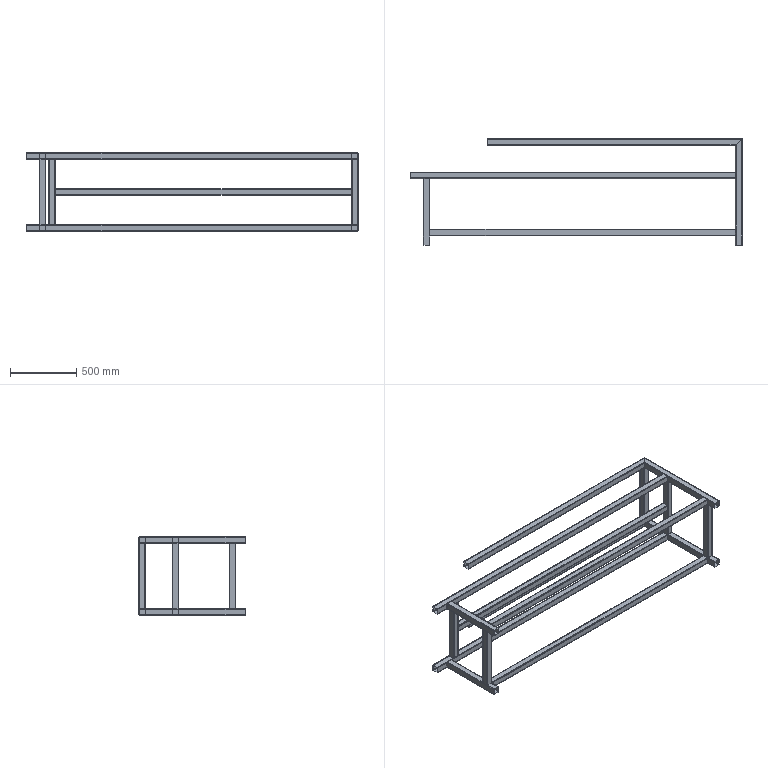Component | SolidWorks | Frame-1 | 16 solids | 288 faces | box 2500 x 800 x 590 mm | volume 9415617 mm3 | plane 160 | cylinder 128 | commonest cylinder face diameters 5 x64 10 x64
build123d program:
from build123d import *

# Parameters (mm, degrees)
SQUARE_TUBE_50_X_50_X_2_5_1_DEPTH     = 526
SQUARE_TUBE_50_X_50_X_2_5_1_2_DEPTH   = 775
SQUARE_TUBE_50_X_50_X_2_5_1_3_DEPTH   = 2352
SQUARE_TUBE_50_X_50_X_2_5_1_4_DEPTH   = 2476
SQUARE_TUBE_50_X_50_X_2_5_2_DEPTH     = 1895
BODY_START                            = 141.421
BODY_5_RUN_ON_DEPTH                   = 166.421
BODY_START_2                          = 633.579
BODY_2_RUN_ON_DEPTH                   = 166.421
SQUARE_TUBE_50_X_50_X_2_5_5_DEPTH     = 526
SQUARE_TUBE_50_X_50_X_2_5_5_2_DEPTH   = 800
SQUARE_TUBE_50_X_50_X_2_5_5_3_DEPTH   = 2352
SQUARE_TUBE_50_X_50_X_2_5_5_4_DEPTH   = 2476
SQUARE_TUBE_50_X_50_X_2_5_5_5_DEPTH   = 1896
BODY_START_3                          = 167.421
BODY_10_RUN_ON_DEPTH                  = 191.421
SQUARE_TUBE_50_X_50_X_2_5_6_DEPTH     = 540
SQUARE_TUBE_50_X_50_X_2_5_6_2_DEPTH   = 540
SQUARE_TUBE_50_X_50_X_2_5_6_3_DEPTH   = 540
SQUARE_TUBE_50_X_50_X_2_5_6_4_DEPTH   = 540
SQUARE_TUBE_50_X_50_X_2_5_6_5_DEPTH   = 540
SQUARE_TUBE_50_X_50_X_2_5_1_2_2_DEPTH = 2277.579


with BuildPart() as part:
    # Sketch1 → Square Tube 50 X 50 X 2.5_1 (new body)
    with BuildSketch(Plane(origin=(0, 0, 0), x_dir=(1, 0, 0), z_dir=(0, 1, 0))):
        with BuildLine():
            Line((-20, -25), (20, -25))
            ThreePointArc((20, -25), (23.536, -23.536), (25, -20))
            Line((25, -20), (25, 20))
            ThreePointArc((25, 20), (23.536, 23.536), (20, 25))
            Line((20, 25), (-20, 25))
            ThreePointArc((-20, 25), (-23.536, 23.536), (-25, 20))
            Line((-25, 20), (-25, -20))
            ThreePointArc((-25, -20), (-23.536, -23.536), (-20, -25))
        make_face()
        with BuildLine():
            Line((-20, -22.5), (20, -22.5))
            ThreePointArc((20, -22.5), (21.768, -21.768), (22.5, -20))
            Line((22.5, -20), (22.5, 20))
            ThreePointArc((22.5, 20), (21.768, 21.768), (20, 22.5))
            Line((20, 22.5), (-20, 22.5))
            ThreePointArc((-20, 22.5), (-21.768, 21.768), (-22.5, 20))
            Line((-22.5, 20), (-22.5, -20))
            ThreePointArc((-22.5, -20), (-21.768, -21.768), (-20, -22.5))
        make_face(mode=Mode.SUBTRACT)
    extrude(amount=SQUARE_TUBE_50_X_50_X_2_5_1_DEPTH)

    # Square Tube 50 X 50 X 2.5_1 end butt 1
    split(bisect_by=Plane.XZ.offset(-500), keep=Keep.TOP)


with BuildPart() as body_2:
    # Sketch1 on segment 2 (on carried to segment 2) → Square Tube 50 X 50 X 2.5_1 2 (new body)
    with BuildSketch(Plane(origin=(2350, 0, 0), x_dir=(1, 0, 0), z_dir=(0, 1, 0))):
        with BuildLine():
            Line((-20, -25), (20, -25))
            ThreePointArc((20, -25), (23.536, -23.536), (25, -20))
            Line((25, -20), (25, 20))
            ThreePointArc((25, 20), (23.536, 23.536), (20, 25))
            Line((20, 25), (-20, 25))
            ThreePointArc((-20, 25), (-23.536, 23.536), (-25, 20))
            Line((-25, 20), (-25, -20))
            ThreePointArc((-25, -20), (-23.536, -23.536), (-20, -25))
        make_face()
        with BuildLine():
            Line((-20, -22.5), (20, -22.5))
            ThreePointArc((20, -22.5), (21.768, -21.768), (22.5, -20))
            Line((22.5, -20), (22.5, 20))
            ThreePointArc((22.5, 20), (21.768, 21.768), (20, 22.5))
            Line((20, 22.5), (-20, 22.5))
            ThreePointArc((-20, 22.5), (-21.768, 21.768), (-22.5, 20))
            Line((-22.5, 20), (-22.5, -20))
            ThreePointArc((-22.5, -20), (-21.768, -21.768), (-20, -22.5))
        make_face(mode=Mode.SUBTRACT)
    extrude(amount=SQUARE_TUBE_50_X_50_X_2_5_1_2_DEPTH)

    # body 2 cut square before the run-on
    split(bisect_by=Plane(origin=(2350, 633.579, 0), x_dir=(1, 0, 0), z_dir=(0, -1, 0)), keep=Keep.TOP)

    # Sketch1 on segment 2 (on carried to segment 2) → body 2 run on (add)
    with BuildSketch(Plane(origin=(2350, 0, 0), x_dir=(1, 0, 0), z_dir=(0, 1, 0)).offset(BODY_START_2)):
        with BuildLine():
            Line((-20, -25), (20, -25))
            ThreePointArc((20, -25), (23.536, -23.536), (25, -20))
            Line((25, -20), (25, 20))
            ThreePointArc((25, 20), (23.536, 23.536), (20, 25))
            Line((20, 25), (-20, 25))
            ThreePointArc((-20, 25), (-23.536, 23.536), (-25, 20))
            Line((-25, 20), (-25, -20))
            ThreePointArc((-25, -20), (-23.536, -23.536), (-20, -25))
        make_face()
        with BuildLine():
            Line((-20, -22.5), (20, -22.5))
            ThreePointArc((20, -22.5), (21.768, -21.768), (22.5, -20))
            Line((22.5, -20), (22.5, 20))
            ThreePointArc((22.5, 20), (21.768, 21.768), (20, 22.5))
            Line((20, 22.5), (-20, 22.5))
            ThreePointArc((-20, 22.5), (-21.768, 21.768), (-22.5, 20))
            Line((-22.5, 20), (-22.5, -20))
            ThreePointArc((-22.5, -20), (-21.768, -21.768), (-20, -22.5))
        make_face(mode=Mode.SUBTRACT)
    extrude(amount=BODY_2_RUN_ON_DEPTH)

    # Trim_Extend1
    split(bisect_by=Plane(origin=(2350, 775, 0), x_dir=(0.7071, 0.7071, 0), z_dir=(0.7071, -0.7071, 0)), keep=Keep.TOP)


with BuildPart() as body_3:
    # Sketch1 on segment 3 (on carried to segment 3) → Square Tube 50 X 50 X 2.5_1 3 (new body)
    with BuildSketch(Plane(origin=(-1, 95, 0), x_dir=(0, -1, 0), z_dir=(1, 0, 0))):
        with BuildLine():
            Line((-20, -25), (20, -25))
            ThreePointArc((20, -25), (23.536, -23.536), (25, -20))
            Line((25, -20), (25, 20))
            ThreePointArc((25, 20), (23.536, 23.536), (20, 25))
            Line((20, 25), (-20, 25))
            ThreePointArc((-20, 25), (-23.536, 23.536), (-25, 20))
            Line((-25, 20), (-25, -20))
            ThreePointArc((-25, -20), (-23.536, -23.536), (-20, -25))
        make_face()
        with BuildLine():
            Line((-20, -22.5), (20, -22.5))
            ThreePointArc((20, -22.5), (21.768, -21.768), (22.5, -20))
            Line((22.5, -20), (22.5, 20))
            ThreePointArc((22.5, 20), (21.768, 21.768), (20, 22.5))
            Line((20, 22.5), (-20, 22.5))
            ThreePointArc((-20, 22.5), (-21.768, 21.768), (-22.5, 20))
            Line((-22.5, 20), (-22.5, -20))
            ThreePointArc((-22.5, -20), (-21.768, -21.768), (-20, -22.5))
        make_face(mode=Mode.SUBTRACT)
    extrude(amount=SQUARE_TUBE_50_X_50_X_2_5_1_3_DEPTH)

    # Square Tube 50 X 50 X 2.5_1 3 end butt 1
    split(bisect_by=Plane(origin=(25, 95, 0), x_dir=(0, 1, 0), z_dir=(1, 0, 0)), keep=Keep.TOP)

    # Square Tube 50 X 50 X 2.5_1 3 end butt 2
    split(bisect_by=Plane(origin=(2325, 95, 0), x_dir=(0, -1, 0), z_dir=(-1, 0, 0)), keep=Keep.TOP)


with BuildPart() as body_4:
    # Sketch1 on segment 4 (on carried to segment 4) → Square Tube 50 X 50 X 2.5_1 4 (new body)
    with BuildSketch(Plane(origin=(-125, 525, 0), x_dir=(0, -1, 0), z_dir=(1, 0, 0))):
        with BuildLine():
            Line((-20, -25), (20, -25))
            ThreePointArc((20, -25), (23.536, -23.536), (25, -20))
            Line((25, -20), (25, 20))
            ThreePointArc((25, 20), (23.536, 23.536), (20, 25))
            Line((20, 25), (-20, 25))
            ThreePointArc((-20, 25), (-23.536, 23.536), (-25, 20))
            Line((-25, 20), (-25, -20))
            ThreePointArc((-25, -20), (-23.536, -23.536), (-20, -25))
        make_face()
        with BuildLine():
            Line((-20, -22.5), (20, -22.5))
            ThreePointArc((20, -22.5), (21.768, -21.768), (22.5, -20))
            Line((22.5, -20), (22.5, 20))
            ThreePointArc((22.5, 20), (21.768, 21.768), (20, 22.5))
            Line((20, 22.5), (-20, 22.5))
            ThreePointArc((-20, 22.5), (-21.768, 21.768), (-22.5, 20))
            Line((-22.5, 20), (-22.5, -20))
            ThreePointArc((-22.5, -20), (-21.768, -21.768), (-20, -22.5))
        make_face(mode=Mode.SUBTRACT)
    extrude(amount=SQUARE_TUBE_50_X_50_X_2_5_1_4_DEPTH)

    # Square Tube 50 X 50 X 2.5_1 4 end butt 1
    split(bisect_by=Plane(origin=(2325, 525, 0), x_dir=(0, -1, 0), z_dir=(-1, 0, 0)), keep=Keep.TOP)


with BuildPart() as body_5:
    # Sketch11 → Square Tube 50 X 50 X 2.5_2 (new body)
    with BuildSketch(Plane(origin=(2350, 775, 0), x_dir=(0, 0, 1), z_dir=(-1, 0, 0))):
        with BuildLine():
            Line((-20, -25), (20, -25))
            ThreePointArc((20, -25), (23.536, -23.536), (25, -20))
            Line((25, -20), (25, 20))
            ThreePointArc((25, 20), (23.536, 23.536), (20, 25))
            Line((20, 25), (-20, 25))
            ThreePointArc((-20, 25), (-23.536, 23.536), (-25, 20))
            Line((-25, 20), (-25, -20))
            ThreePointArc((-25, -20), (-23.536, -23.536), (-20, -25))
        make_face()
        with BuildLine():
            Line((-20, -22.5), (20, -22.5))
            ThreePointArc((20, -22.5), (21.768, -21.768), (22.5, -20))
            Line((22.5, -20), (22.5, 20))
            ThreePointArc((22.5, 20), (21.768, 21.768), (20, 22.5))
            Line((20, 22.5), (-20, 22.5))
            ThreePointArc((-20, 22.5), (-21.768, 21.768), (-22.5, 20))
            Line((-22.5, 20), (-22.5, -20))
            ThreePointArc((-22.5, -20), (-21.768, -21.768), (-20, -22.5))
        make_face(mode=Mode.SUBTRACT)
    extrude(amount=SQUARE_TUBE_50_X_50_X_2_5_2_DEPTH)

    # body 5 cut square before the run-on
    split(bisect_by=Plane(origin=(2208.579, 775, 0), x_dir=(0, -1, 0), z_dir=(-1, 0, 0)), keep=Keep.TOP)

    # Sketch11 → body 5 run on (add)
    with BuildSketch(Plane(origin=(2350, 775, 0), x_dir=(0, 0, 1), z_dir=(-1, 0, 0)).offset(BODY_START)):
        with BuildLine():
            Line((-20, -25), (20, -25))
            ThreePointArc((20, -25), (23.536, -23.536), (25, -20))
            Line((25, -20), (25, 20))
            ThreePointArc((25, 20), (23.536, 23.536), (20, 25))
            Line((20, 25), (-20, 25))
            ThreePointArc((-20, 25), (-23.536, 23.536), (-25, 20))
            Line((-25, 20), (-25, -20))
            ThreePointArc((-25, -20), (-23.536, -23.536), (-20, -25))
        make_face()
        with BuildLine():
            Line((-20, -22.5), (20, -22.5))
            ThreePointArc((20, -22.5), (21.768, -21.768), (22.5, -20))
            Line((22.5, -20), (22.5, 20))
            ThreePointArc((22.5, 20), (21.768, 21.768), (20, 22.5))
            Line((20, 22.5), (-20, 22.5))
            ThreePointArc((-20, 22.5), (-21.768, 21.768), (-22.5, 20))
            Line((-22.5, 20), (-22.5, -20))
            ThreePointArc((-22.5, -20), (-21.768, -21.768), (-20, -22.5))
        make_face(mode=Mode.SUBTRACT)
    extrude(amount=-BODY_5_RUN_ON_DEPTH)

    # Trim_Extend1
    split(bisect_by=Plane(origin=(2350, 775, 0), x_dir=(-0.7071, -0.7071, 0), z_dir=(-0.7071, 0.7071, 0)), keep=Keep.TOP)


with BuildPart() as body_6:
    # Sketch12 → Square Tube 50 X 50 X 2.5_5 (new body)
    with BuildSketch(Plane(origin=(0, 0, 540), x_dir=(-1, 0, 0), z_dir=(0, 1, 0))):
        with BuildLine():
            Line((-20, -25), (20, -25))
            ThreePointArc((20, -25), (23.536, -23.536), (25, -20))
            Line((25, -20), (25, 20))
            ThreePointArc((25, 20), (23.536, 23.536), (20, 25))
            Line((20, 25), (-20, 25))
            ThreePointArc((-20, 25), (-23.536, 23.536), (-25, 20))
            Line((-25, 20), (-25, -20))
            ThreePointArc((-25, -20), (-23.536, -23.536), (-20, -25))
        make_face()
        with BuildLine():
            Line((-20, -22.5), (20, -22.5))
            ThreePointArc((20, -22.5), (21.768, -21.768), (22.5, -20))
            Line((22.5, -20), (22.5, 20))
            ThreePointArc((22.5, 20), (21.768, 21.768), (20, 22.5))
            Line((20, 22.5), (-20, 22.5))
            ThreePointArc((-20, 22.5), (-21.768, 21.768), (-22.5, 20))
            Line((-22.5, 20), (-22.5, -20))
            ThreePointArc((-22.5, -20), (-21.768, -21.768), (-20, -22.5))
        make_face(mode=Mode.SUBTRACT)
    extrude(amount=SQUARE_TUBE_50_X_50_X_2_5_5_DEPTH)

    # Square Tube 50 X 50 X 2.5_5 end butt 1
    split(bisect_by=Plane(origin=(0, 500, 540), x_dir=(1, 0, 0), z_dir=(0, -1, 0)), keep=Keep.TOP)


with BuildPart() as body_7:
    # Sketch12 on segment 2 (on carried to segment 2) → Square Tube 50 X 50 X 2.5_5 2 (new body)
    with BuildSketch(Plane(origin=(2350, 0, 540), x_dir=(-1, 0, 0), z_dir=(0, 1, 0))):
        with BuildLine():
            Line((-20, -25), (20, -25))
            ThreePointArc((20, -25), (23.536, -23.536), (25, -20))
            Line((25, -20), (25, 20))
            ThreePointArc((25, 20), (23.536, 23.536), (20, 25))
            Line((20, 25), (-20, 25))
            ThreePointArc((-20, 25), (-23.536, 23.536), (-25, 20))
            Line((-25, 20), (-25, -20))
            ThreePointArc((-25, -20), (-23.536, -23.536), (-20, -25))
        make_face()
        with BuildLine():
            Line((-20, -22.5), (20, -22.5))
            ThreePointArc((20, -22.5), (21.768, -21.768), (22.5, -20))
            Line((22.5, -20), (22.5, 20))
            ThreePointArc((22.5, 20), (21.768, 21.768), (20, 22.5))
            Line((20, 22.5), (-20, 22.5))
            ThreePointArc((-20, 22.5), (-21.768, 21.768), (-22.5, 20))
            Line((-22.5, 20), (-22.5, -20))
            ThreePointArc((-22.5, -20), (-21.768, -21.768), (-20, -22.5))
        make_face(mode=Mode.SUBTRACT)
    extrude(amount=SQUARE_TUBE_50_X_50_X_2_5_5_2_DEPTH)

    # Trim_Extend2
    split(bisect_by=Plane(origin=(2350, 775, 540), x_dir=(0.7071, 0.7071, 0), z_dir=(0.7071, -0.7071, 0)), keep=Keep.TOP)


with BuildPart() as body_8:
    # Sketch12 on segment 3 (on carried to segment 3) → Square Tube 50 X 50 X 2.5_5 3 (new body)
    with BuildSketch(Plane(origin=(-1, 95, 540), x_dir=(0, 1, 0), z_dir=(1, 0, 0))):
        with BuildLine():
            Line((-20, -25), (20, -25))
            ThreePointArc((20, -25), (23.536, -23.536), (25, -20))
            Line((25, -20), (25, 20))
            ThreePointArc((25, 20), (23.536, 23.536), (20, 25))
            Line((20, 25), (-20, 25))
            ThreePointArc((-20, 25), (-23.536, 23.536), (-25, 20))
            Line((-25, 20), (-25, -20))
            ThreePointArc((-25, -20), (-23.536, -23.536), (-20, -25))
        make_face()
        with BuildLine():
            Line((-20, -22.5), (20, -22.5))
            ThreePointArc((20, -22.5), (21.768, -21.768), (22.5, -20))
            Line((22.5, -20), (22.5, 20))
            ThreePointArc((22.5, 20), (21.768, 21.768), (20, 22.5))
            Line((20, 22.5), (-20, 22.5))
            ThreePointArc((-20, 22.5), (-21.768, 21.768), (-22.5, 20))
            Line((-22.5, 20), (-22.5, -20))
            ThreePointArc((-22.5, -20), (-21.768, -21.768), (-20, -22.5))
        make_face(mode=Mode.SUBTRACT)
    extrude(amount=SQUARE_TUBE_50_X_50_X_2_5_5_3_DEPTH)

    # Square Tube 50 X 50 X 2.5_5 3 end butt 1
    split(bisect_by=Plane(origin=(25, 95, 540), x_dir=(0, 1, 0), z_dir=(1, 0, 0)), keep=Keep.TOP)

    # Square Tube 50 X 50 X 2.5_5 3 end butt 2
    split(bisect_by=Plane(origin=(2325, 95, 540), x_dir=(0, -1, 0), z_dir=(-1, 0, 0)), keep=Keep.TOP)


with BuildPart() as body_9:
    # Sketch12 on segment 4 (on carried to segment 4) → Square Tube 50 X 50 X 2.5_5 4 (new body)
    with BuildSketch(Plane(origin=(-125, 525, 540), x_dir=(0, 1, 0), z_dir=(1, 0, 0))):
        with BuildLine():
            Line((-20, -25), (20, -25))
            ThreePointArc((20, -25), (23.536, -23.536), (25, -20))
            Line((25, -20), (25, 20))
            ThreePointArc((25, 20), (23.536, 23.536), (20, 25))
            Line((20, 25), (-20, 25))
            ThreePointArc((-20, 25), (-23.536, 23.536), (-25, 20))
            Line((-25, 20), (-25, -20))
            ThreePointArc((-25, -20), (-23.536, -23.536), (-20, -25))
        make_face()
        with BuildLine():
            Line((-20, -22.5), (20, -22.5))
            ThreePointArc((20, -22.5), (21.768, -21.768), (22.5, -20))
            Line((22.5, -20), (22.5, 20))
            ThreePointArc((22.5, 20), (21.768, 21.768), (20, 22.5))
            Line((20, 22.5), (-20, 22.5))
            ThreePointArc((-20, 22.5), (-21.768, 21.768), (-22.5, 20))
            Line((-22.5, 20), (-22.5, -20))
            ThreePointArc((-22.5, -20), (-21.768, -21.768), (-20, -22.5))
        make_face(mode=Mode.SUBTRACT)
    extrude(amount=SQUARE_TUBE_50_X_50_X_2_5_5_4_DEPTH)

    # Square Tube 50 X 50 X 2.5_5 4 end butt 1
    split(bisect_by=Plane(origin=(2325, 525, 540), x_dir=(0, -1, 0), z_dir=(-1, 0, 0)), keep=Keep.TOP)


with BuildPart() as body_10:
    # Sketch12 on segment 5 (on carried to segment 5) → Square Tube 50 X 50 X 2.5_5 5 (new body)
    with BuildSketch(Plane(origin=(2351, 775, 540), x_dir=(0, -1, 0), z_dir=(-1, 0, 0))):
        with BuildLine():
            Line((-20, -25), (20, -25))
            ThreePointArc((20, -25), (23.536, -23.536), (25, -20))
            Line((25, -20), (25, 20))
            ThreePointArc((25, 20), (23.536, 23.536), (20, 25))
            Line((20, 25), (-20, 25))
            ThreePointArc((-20, 25), (-23.536, 23.536), (-25, 20))
            Line((-25, 20), (-25, -20))
            ThreePointArc((-25, -20), (-23.536, -23.536), (-20, -25))
        make_face()
        with BuildLine():
            Line((-20, -22.5), (20, -22.5))
            ThreePointArc((20, -22.5), (21.768, -21.768), (22.5, -20))
            Line((22.5, -20), (22.5, 20))
            ThreePointArc((22.5, 20), (21.768, 21.768), (20, 22.5))
            Line((20, 22.5), (-20, 22.5))
            ThreePointArc((-20, 22.5), (-21.768, 21.768), (-22.5, 20))
            Line((-22.5, 20), (-22.5, -20))
            ThreePointArc((-22.5, -20), (-21.768, -21.768), (-20, -22.5))
        make_face(mode=Mode.SUBTRACT)
    extrude(amount=SQUARE_TUBE_50_X_50_X_2_5_5_5_DEPTH)

    # Square Tube 50 X 50 X 2.5_5 5 end butt 1
    split(bisect_by=Plane(origin=(2325, 775, 540), x_dir=(0, -1, 0), z_dir=(-1, 0, 0)), keep=Keep.TOP)

    # body 10 cut square before the run-on
    split(bisect_by=Plane(origin=(2183.579, 775, 540), x_dir=(0, -1, 0), z_dir=(-1, 0, 0)), keep=Keep.TOP)

    # Sketch12 on segment 5 (on carried to segment 5) → body 10 run on (add)
    with BuildSketch(Plane(origin=(2351, 775, 540), x_dir=(0, -1, 0), z_dir=(-1, 0, 0)).offset(BODY_START_3)):
        with BuildLine():
            Line((-20, -25), (20, -25))
            ThreePointArc((20, -25), (23.536, -23.536), (25, -20))
            Line((25, -20), (25, 20))
            ThreePointArc((25, 20), (23.536, 23.536), (20, 25))
            Line((20, 25), (-20, 25))
            ThreePointArc((-20, 25), (-23.536, 23.536), (-25, 20))
            Line((-25, 20), (-25, -20))
            ThreePointArc((-25, -20), (-23.536, -23.536), (-20, -25))
        make_face()
        with BuildLine():
            Line((-20, -22.5), (20, -22.5))
            ThreePointArc((20, -22.5), (21.768, -21.768), (22.5, -20))
            Line((22.5, -20), (22.5, 20))
            ThreePointArc((22.5, 20), (21.768, 21.768), (20, 22.5))
            Line((20, 22.5), (-20, 22.5))
            ThreePointArc((-20, 22.5), (-21.768, 21.768), (-22.5, 20))
            Line((-22.5, 20), (-22.5, -20))
            ThreePointArc((-22.5, -20), (-21.768, -21.768), (-20, -22.5))
        make_face(mode=Mode.SUBTRACT)
    extrude(amount=-BODY_10_RUN_ON_DEPTH)

    # Trim_Extend2
    split(bisect_by=Plane(origin=(2350, 775, 540), x_dir=(-0.7071, -0.7071, 0), z_dir=(-0.7071, 0.7071, 0)), keep=Keep.TOP)


with BuildPart() as body_11:
    # Sketch13 → Square Tube 50 X 50 X 2.5_6 (new body)
    with BuildSketch(Plane(origin=(72.421, 525, 540), x_dir=(1, 0, 0), z_dir=(0, 0, -1))):
        with BuildLine():
            Line((-20, -25), (20, -25))
            ThreePointArc((20, -25), (23.536, -23.536), (25, -20))
            Line((25, -20), (25, 20))
            ThreePointArc((25, 20), (23.536, 23.536), (20, 25))
            Line((20, 25), (-20, 25))
            ThreePointArc((-20, 25), (-23.536, 23.536), (-25, 20))
            Line((-25, 20), (-25, -20))
            ThreePointArc((-25, -20), (-23.536, -23.536), (-20, -25))
        make_face()
        with BuildLine():
            Line((-20, -22.5), (20, -22.5))
            ThreePointArc((20, -22.5), (21.768, -21.768), (22.5, -20))
            Line((22.5, -20), (22.5, 20))
            ThreePointArc((22.5, 20), (21.768, 21.768), (20, 22.5))
            Line((20, 22.5), (-20, 22.5))
            ThreePointArc((-20, 22.5), (-21.768, 21.768), (-22.5, 20))
            Line((-22.5, 20), (-22.5, -20))
            ThreePointArc((-22.5, -20), (-21.768, -21.768), (-20, -22.5))
        make_face(mode=Mode.SUBTRACT)
    extrude(amount=SQUARE_TUBE_50_X_50_X_2_5_6_DEPTH)

    # Trim_Extend3
    split(bisect_by=Plane(origin=(0, 250, 25), x_dir=(0, -1, 0), z_dir=(0, 0, 1)), keep=Keep.TOP)

    # Trim_Extend4
    split(bisect_by=Plane(origin=(1175, 95, 515), x_dir=(0, 1, 0), z_dir=(0, 0, -1)), keep=Keep.TOP)


with BuildPart() as body_12:
    # Sketch13 on segment 2 (on carried to segment 2) → Square Tube 50 X 50 X 2.5_6 2 (new body)
    with BuildSketch(Plane(origin=(0, 95, 540), x_dir=(1, 0, 0), z_dir=(0, 0, -1))):
        with BuildLine():
            Line((-20, -25), (20, -25))
            ThreePointArc((20, -25), (23.536, -23.536), (25, -20))
            Line((25, -20), (25, 20))
            ThreePointArc((25, 20), (23.536, 23.536), (20, 25))
            Line((20, 25), (-20, 25))
            ThreePointArc((-20, 25), (-23.536, 23.536), (-25, 20))
            Line((-25, 20), (-25, -20))
            ThreePointArc((-25, -20), (-23.536, -23.536), (-20, -25))
        make_face()
        with BuildLine():
            Line((-20, -22.5), (20, -22.5))
            ThreePointArc((20, -22.5), (21.768, -21.768), (22.5, -20))
            Line((22.5, -20), (22.5, 20))
            ThreePointArc((22.5, 20), (21.768, 21.768), (20, 22.5))
            Line((20, 22.5), (-20, 22.5))
            ThreePointArc((-20, 22.5), (-21.768, 21.768), (-22.5, 20))
            Line((-22.5, 20), (-22.5, -20))
            ThreePointArc((-22.5, -20), (-21.768, -21.768), (-20, -22.5))
        make_face(mode=Mode.SUBTRACT)
    extrude(amount=SQUARE_TUBE_50_X_50_X_2_5_6_2_DEPTH)

    # Trim_Extend3
    split(bisect_by=Plane(origin=(0, 250, 25), x_dir=(0, -1, 0), z_dir=(0, 0, 1)), keep=Keep.TOP)

    # Trim_Extend4
    split(bisect_by=Plane(origin=(1175, 95, 515), x_dir=(0, 1, 0), z_dir=(0, 0, -1)), keep=Keep.TOP)


with BuildPart() as body_13:
    # Sketch13 on segment 3 (on carried to segment 3) → Square Tube 50 X 50 X 2.5_6 3 (new body)
    with BuildSketch(Plane(origin=(2350, 95, 540), x_dir=(1, 0, 0), z_dir=(0, 0, -1))):
        with BuildLine():
            Line((-20, -25), (20, -25))
            ThreePointArc((20, -25), (23.536, -23.536), (25, -20))
            Line((25, -20), (25, 20))
            ThreePointArc((25, 20), (23.536, 23.536), (20, 25))
            Line((20, 25), (-20, 25))
            ThreePointArc((-20, 25), (-23.536, 23.536), (-25, 20))
            Line((-25, 20), (-25, -20))
            ThreePointArc((-25, -20), (-23.536, -23.536), (-20, -25))
        make_face()
        with BuildLine():
            Line((-20, -22.5), (20, -22.5))
            ThreePointArc((20, -22.5), (21.768, -21.768), (22.5, -20))
            Line((22.5, -20), (22.5, 20))
            ThreePointArc((22.5, 20), (21.768, 21.768), (20, 22.5))
            Line((20, 22.5), (-20, 22.5))
            ThreePointArc((-20, 22.5), (-21.768, 21.768), (-22.5, 20))
            Line((-22.5, 20), (-22.5, -20))
            ThreePointArc((-22.5, -20), (-21.768, -21.768), (-20, -22.5))
        make_face(mode=Mode.SUBTRACT)
    extrude(amount=SQUARE_TUBE_50_X_50_X_2_5_6_3_DEPTH)

    # Trim_Extend3
    split(bisect_by=Plane(origin=(0, 250, 25), x_dir=(0, -1, 0), z_dir=(0, 0, 1)), keep=Keep.TOP)

    # Trim_Extend4
    split(bisect_by=Plane(origin=(1175, 95, 515), x_dir=(0, 1, 0), z_dir=(0, 0, -1)), keep=Keep.TOP)


with BuildPart() as body_14:
    # Sketch13 on segment 4 (on carried to segment 4) → Square Tube 50 X 50 X 2.5_6 4 (new body)
    with BuildSketch(Plane(origin=(2350, 525, 540), x_dir=(1, 0, 0), z_dir=(0, 0, -1))):
        with BuildLine():
            Line((-20, -25), (20, -25))
            ThreePointArc((20, -25), (23.536, -23.536), (25, -20))
            Line((25, -20), (25, 20))
            ThreePointArc((25, 20), (23.536, 23.536), (20, 25))
            Line((20, 25), (-20, 25))
            ThreePointArc((-20, 25), (-23.536, 23.536), (-25, 20))
            Line((-25, 20), (-25, -20))
            ThreePointArc((-25, -20), (-23.536, -23.536), (-20, -25))
        make_face()
        with BuildLine():
            Line((-20, -22.5), (20, -22.5))
            ThreePointArc((20, -22.5), (21.768, -21.768), (22.5, -20))
            Line((22.5, -20), (22.5, 20))
            ThreePointArc((22.5, 20), (21.768, 21.768), (20, 22.5))
            Line((20, 22.5), (-20, 22.5))
            ThreePointArc((-20, 22.5), (-21.768, 21.768), (-22.5, 20))
            Line((-22.5, 20), (-22.5, -20))
            ThreePointArc((-22.5, -20), (-21.768, -21.768), (-20, -22.5))
        make_face(mode=Mode.SUBTRACT)
    extrude(amount=SQUARE_TUBE_50_X_50_X_2_5_6_4_DEPTH)

    # Trim_Extend3
    split(bisect_by=Plane(origin=(0, 250, 25), x_dir=(0, -1, 0), z_dir=(0, 0, 1)), keep=Keep.TOP)

    # Trim_Extend4
    split(bisect_by=Plane(origin=(1175, 95, 515), x_dir=(0, 1, 0), z_dir=(0, 0, -1)), keep=Keep.TOP)


with BuildPart() as body_15:
    # Sketch13 on segment 5 (on carried to segment 5) → Square Tube 50 X 50 X 2.5_6 5 (new body)
    with BuildSketch(Plane(origin=(2350, 775, 540), x_dir=(1, 0, 0), z_dir=(0, 0, -1))):
        with BuildLine():
            Line((-20, -25), (20, -25))
            ThreePointArc((20, -25), (23.536, -23.536), (25, -20))
            Line((25, -20), (25, 20))
            ThreePointArc((25, 20), (23.536, 23.536), (20, 25))
            Line((20, 25), (-20, 25))
            ThreePointArc((-20, 25), (-23.536, 23.536), (-25, 20))
            Line((-25, 20), (-25, -20))
            ThreePointArc((-25, -20), (-23.536, -23.536), (-20, -25))
        make_face()
        with BuildLine():
            Line((-20, -22.5), (20, -22.5))
            ThreePointArc((20, -22.5), (21.768, -21.768), (22.5, -20))
            Line((22.5, -20), (22.5, 20))
            ThreePointArc((22.5, 20), (21.768, 21.768), (20, 22.5))
            Line((20, 22.5), (-20, 22.5))
            ThreePointArc((-20, 22.5), (-21.768, 21.768), (-22.5, 20))
            Line((-22.5, 20), (-22.5, -20))
            ThreePointArc((-22.5, -20), (-21.768, -21.768), (-20, -22.5))
        make_face(mode=Mode.SUBTRACT)
    extrude(amount=SQUARE_TUBE_50_X_50_X_2_5_6_5_DEPTH)

    # Trim_Extend3
    split(bisect_by=Plane(origin=(0, 250, 25), x_dir=(0, -1, 0), z_dir=(0, 0, 1)), keep=Keep.TOP)

    # Trim_Extend4
    split(bisect_by=Plane(origin=(1175, 95, 515), x_dir=(0, 1, 0), z_dir=(0, 0, -1)), keep=Keep.TOP)


with BuildPart() as body_16:
    # Sketch14 → Square Tube 50 X 50 X 2.5_1__2 2 (new body)
    with BuildSketch(Plane(origin=(72.421, 525, 270), x_dir=(0, 0, -1), z_dir=(1, 0, 0))):
        with BuildLine():
            Line((-20, -25), (20, -25))
            ThreePointArc((20, -25), (23.536, -23.536), (25, -20))
            Line((25, -20), (25, 20))
            ThreePointArc((25, 20), (23.536, 23.536), (20, 25))
            Line((20, 25), (-20, 25))
            ThreePointArc((-20, 25), (-23.536, 23.536), (-25, 20))
            Line((-25, 20), (-25, -20))
            ThreePointArc((-25, -20), (-23.536, -23.536), (-20, -25))
        make_face()
        with BuildLine():
            Line((-20, -22.5), (20, -22.5))
            ThreePointArc((20, -22.5), (21.768, -21.768), (22.5, -20))
            Line((22.5, -20), (22.5, 20))
            ThreePointArc((22.5, 20), (21.768, 21.768), (20, 22.5))
            Line((20, 22.5), (-20, 22.5))
            ThreePointArc((-20, 22.5), (-21.768, 21.768), (-22.5, 20))
            Line((-22.5, 20), (-22.5, -20))
            ThreePointArc((-22.5, -20), (-21.768, -21.768), (-20, -22.5))
        make_face(mode=Mode.SUBTRACT)
    extrude(amount=SQUARE_TUBE_50_X_50_X_2_5_1_2_2_DEPTH)

    # Trim_Extend5
    split(bisect_by=Plane(origin=(97.421, 525, 270), x_dir=(0, 1, 0), z_dir=(1, 0, 0)), keep=Keep.TOP)

    # Trim_Extend5 3
    split(bisect_by=Plane(origin=(2325, 525, 270), x_dir=(0, -1, 0), z_dir=(-1, 0, 0)), keep=Keep.TOP)


solid = Compound([part.part, body_2.part, body_3.part, body_4.part, body_5.part, body_6.part, body_7.part, body_8.part, body_9.part, body_10.part, body_11.part, body_12.part, body_13.part, body_14.part, body_15.part, body_16.part])